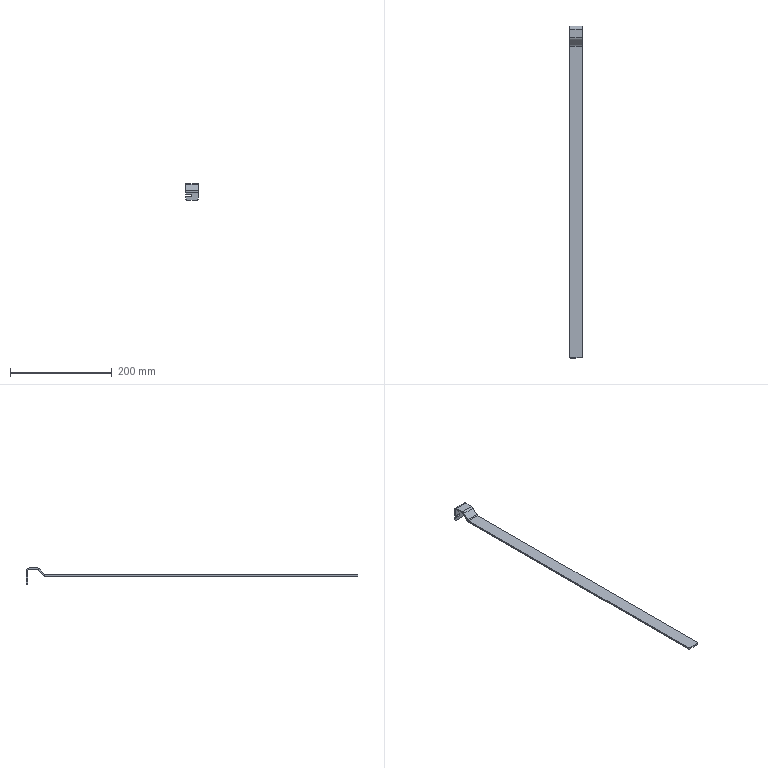Component | SolidWorks | PC-CAJ-P08-1_PM-CAJ-P61-1 | 1 solid | 38 faces | box 25.4 x 651.9 x 31.5 mm | volume 54906 mm3 | plane 28 | cylinder 10 | commonest cylinder face diameters 4 x4 12.7 x3 6.35 x3 | material Plain Carbon Steel
STEP:
#1=COLOUR_RGB('',0.7922,0.8196,0.9333);
#2=FILL_AREA_STYLE_COLOUR('',#1);
#3=FILL_AREA_STYLE('',(#2));
#4=SURFACE_STYLE_FILL_AREA(#3);
#5=SURFACE_SIDE_STYLE('',(#4));
#6=SURFACE_STYLE_USAGE(.BOTH.,#5);
#7=PRESENTATION_STYLE_ASSIGNMENT((#6));
#8=CARTESIAN_POINT('',(0.4213,-26.5,8.548));
#9=VERTEX_POINT('',#8);
#10=CARTESIAN_POINT('',(0.5,-26.421,8.548));
#11=VERTEX_POINT('',#10);
#12=CARTESIAN_POINT('',(0.4213,-26.421,8.548));
#13=DIRECTION('',(0.,0.,1.));
#14=DIRECTION('',(-1.,0.,0.));
#15=AXIS2_PLACEMENT_3D('',#12,#13,#14);
#16=CIRCLE('',#15,0.07874);
#17=EDGE_CURVE('',#9,#11,#16,.T.);
#18=ORIENTED_EDGE('',*,*,#17,.T.);
#19=CARTESIAN_POINT('',(0.5,-26.421,8.673));
#20=VERTEX_POINT('',#19);
#21=CARTESIAN_POINT('',(0.5,-26.421,8.611));
#22=DIRECTION('',(-0.,0.,1.));
#23=VECTOR('',#22,39.37);
#24=LINE('',#21,#23);
#25=EDGE_CURVE('',#11,#20,#24,.T.);
#26=ORIENTED_EDGE('',*,*,#25,.T.);
#27=CARTESIAN_POINT('',(0.4213,-26.5,8.673));
#28=VERTEX_POINT('',#27);
#29=CARTESIAN_POINT('',(0.4213,-26.421,8.673));
#30=DIRECTION('',(-0.,-0.,-1.));
#31=DIRECTION('',(-1.,0.,0.));
#32=AXIS2_PLACEMENT_3D('',#29,#30,#31);
#33=CIRCLE('',#32,0.07874);
#34=EDGE_CURVE('',#20,#28,#33,.T.);
#35=ORIENTED_EDGE('',*,*,#34,.T.);
#36=CARTESIAN_POINT('',(0.4213,-26.5,8.611));
#37=DIRECTION('',(0.,-0.,-1.));
#38=VECTOR('',#37,39.37);
#39=LINE('',#36,#38);
#40=EDGE_CURVE('',#28,#9,#39,.T.);
#41=ORIENTED_EDGE('',*,*,#40,.T.);
#42=EDGE_LOOP('',(#18,#26,#35,#41));
#43=FACE_OUTER_BOUND('',#42,.T.);
#44=CARTESIAN_POINT('',(0.4213,-26.421,8.673));
#45=DIRECTION('',(-0.,-0.,-1.));
#46=DIRECTION('',(-1.,0.,0.));
#47=AXIS2_PLACEMENT_3D('',#44,#45,#46);
#48=CYLINDRICAL_SURFACE('',#47,0.07874);
#49=ADVANCED_FACE('',(#43),#48,.T.);
#50=CARTESIAN_POINT('',(0.5,-2.391,8.548));
#51=VERTEX_POINT('',#50);
#52=CARTESIAN_POINT('',(0.5,-2.391,8.673));
#53=VERTEX_POINT('',#52);
#54=CARTESIAN_POINT('',(0.5,-2.391,8.611));
#55=DIRECTION('',(-0.,0.,1.));
#56=VECTOR('',#55,39.37);
#57=LINE('',#54,#56);
#58=EDGE_CURVE('',#51,#53,#57,.T.);
#59=ORIENTED_EDGE('',*,*,#58,.T.);
#60=CARTESIAN_POINT('',(0.5,-14.406,8.673));
#61=DIRECTION('',(-0.,-1.,0.));
#62=VECTOR('',#61,39.37);
#63=LINE('',#60,#62);
#64=EDGE_CURVE('',#53,#20,#63,.T.);
#65=ORIENTED_EDGE('',*,*,#64,.T.);
#66=ORIENTED_EDGE('',*,*,#25,.F.);
#67=CARTESIAN_POINT('',(0.5,-14.406,8.548));
#68=DIRECTION('',(0.,1.,-0.));
#69=VECTOR('',#68,39.37);
#70=LINE('',#67,#69);
#71=EDGE_CURVE('',#11,#51,#70,.T.);
#72=ORIENTED_EDGE('',*,*,#71,.T.);
#73=EDGE_LOOP('',(#59,#65,#66,#72));
#74=FACE_OUTER_BOUND('',#73,.T.);
#75=CARTESIAN_POINT('',(0.5,-26.421,8.673));
#76=DIRECTION('',(1.,-0.,0.));
#77=DIRECTION('',(0.,-0.,-1.));
#78=AXIS2_PLACEMENT_3D('',#75,#76,#77);
#79=PLANE('',#78);
#80=ADVANCED_FACE('',(#74),#79,.T.);
#81=CARTESIAN_POINT('',(-0.5,-2.391,8.548));
#82=VERTEX_POINT('',#81);
#83=CARTESIAN_POINT('',(0.,-2.391,8.548));
#84=DIRECTION('',(1.,-0.,0.));
#85=VECTOR('',#84,39.37);
#86=LINE('',#83,#85);
#87=EDGE_CURVE('',#82,#51,#86,.T.);
#88=ORIENTED_EDGE('',*,*,#87,.T.);
#89=ORIENTED_EDGE('',*,*,#71,.F.);
#90=ORIENTED_EDGE('',*,*,#17,.F.);
#91=CARTESIAN_POINT('',(-0.4213,-26.5,8.548));
#92=VERTEX_POINT('',#91);
#93=CARTESIAN_POINT('',(-0.,-26.5,8.548));
#94=DIRECTION('',(-1.,0.,-0.));
#95=VECTOR('',#94,39.37);
#96=LINE('',#93,#95);
#97=EDGE_CURVE('',#9,#92,#96,.T.);
#98=ORIENTED_EDGE('',*,*,#97,.T.);
#99=CARTESIAN_POINT('',(-0.5,-26.421,8.548));
#100=VERTEX_POINT('',#99);
#101=CARTESIAN_POINT('',(-0.4213,-26.421,8.548));
#102=DIRECTION('',(0.,-0.,-1.));
#103=DIRECTION('',(-0.,-1.,0.));
#104=AXIS2_PLACEMENT_3D('',#101,#102,#103);
#105=CIRCLE('',#104,0.07874);
#106=EDGE_CURVE('',#92,#100,#105,.T.);
#107=ORIENTED_EDGE('',*,*,#106,.T.);
#108=CARTESIAN_POINT('',(-0.5,-14.445,8.548));
#109=DIRECTION('',(0.,1.,-0.));
#110=VECTOR('',#109,39.37);
#111=LINE('',#108,#110);
#112=EDGE_CURVE('',#100,#82,#111,.T.);
#113=ORIENTED_EDGE('',*,*,#112,.T.);
#114=EDGE_LOOP('',(#88,#89,#90,#98,#107,#113));
#115=FACE_OUTER_BOUND('',#114,.T.);
#116=CARTESIAN_POINT('',(0.5,-2.391,8.548));
#117=DIRECTION('',(0.,-0.,-1.));
#118=DIRECTION('',(-0.,-1.,0.));
#119=AXIS2_PLACEMENT_3D('',#116,#117,#118);
#120=PLANE('',#119);
#121=ADVANCED_FACE('',(#115),#120,.T.);
#122=CARTESIAN_POINT('',(-0.4213,-26.5,8.673));
#123=VERTEX_POINT('',#122);
#124=CARTESIAN_POINT('',(-0.4213,-26.5,8.611));
#125=DIRECTION('',(0.,-0.,-1.));
#126=VECTOR('',#125,39.37);
#127=LINE('',#124,#126);
#128=EDGE_CURVE('',#123,#92,#127,.T.);
#129=ORIENTED_EDGE('',*,*,#128,.T.);
#130=ORIENTED_EDGE('',*,*,#97,.F.);
#131=ORIENTED_EDGE('',*,*,#40,.F.);
#132=CARTESIAN_POINT('',(-0.,-26.5,8.673));
#133=DIRECTION('',(-1.,0.,-0.));
#134=VECTOR('',#133,39.37);
#135=LINE('',#132,#134);
#136=EDGE_CURVE('',#28,#123,#135,.T.);
#137=ORIENTED_EDGE('',*,*,#136,.T.);
#138=EDGE_LOOP('',(#129,#130,#131,#137));
#139=FACE_OUTER_BOUND('',#138,.T.);
#140=CARTESIAN_POINT('',(0.4213,-26.5,8.548));
#141=DIRECTION('',(-0.,-1.,0.));
#142=DIRECTION('',(-0.,0.,1.));
#143=AXIS2_PLACEMENT_3D('',#140,#141,#142);
#144=PLANE('',#143);
#145=ADVANCED_FACE('',(#139),#144,.T.);
#146=CARTESIAN_POINT('',(-0.5,-26.421,8.673));
#147=VERTEX_POINT('',#146);
#148=CARTESIAN_POINT('',(-0.4213,-26.421,8.673));
#149=DIRECTION('',(-0.,0.,1.));
#150=DIRECTION('',(-0.,-1.,0.));
#151=AXIS2_PLACEMENT_3D('',#148,#149,#150);
#152=CIRCLE('',#151,0.07874);
#153=EDGE_CURVE('',#147,#123,#152,.T.);
#154=ORIENTED_EDGE('',*,*,#153,.T.);
#155=ORIENTED_EDGE('',*,*,#136,.F.);
#156=ORIENTED_EDGE('',*,*,#34,.F.);
#157=ORIENTED_EDGE('',*,*,#64,.F.);
#158=CARTESIAN_POINT('',(-0.5,-2.391,8.673));
#159=VERTEX_POINT('',#158);
#160=CARTESIAN_POINT('',(0.,-2.391,8.673));
#161=DIRECTION('',(-1.,0.,-0.));
#162=VECTOR('',#161,39.37);
#163=LINE('',#160,#162);
#164=EDGE_CURVE('',#53,#159,#163,.T.);
#165=ORIENTED_EDGE('',*,*,#164,.T.);
#166=CARTESIAN_POINT('',(-0.5,-14.445,8.673));
#167=DIRECTION('',(-0.,-1.,0.));
#168=VECTOR('',#167,39.37);
#169=LINE('',#166,#168);
#170=EDGE_CURVE('',#159,#147,#169,.T.);
#171=ORIENTED_EDGE('',*,*,#170,.T.);
#172=EDGE_LOOP('',(#154,#155,#156,#157,#165,#171));
#173=FACE_OUTER_BOUND('',#172,.T.);
#174=CARTESIAN_POINT('',(0.5,-26.5,8.673));
#175=DIRECTION('',(-0.,0.,1.));
#176=DIRECTION('',(0.,1.,-0.));
#177=AXIS2_PLACEMENT_3D('',#174,#175,#176);
#178=PLANE('',#177);
#179=ADVANCED_FACE('',(#173),#178,.T.);
#180=ORIENTED_EDGE('',*,*,#58,.F.);
#181=CARTESIAN_POINT('',(0.5,-2.214,8.621));
#182=VERTEX_POINT('',#181);
#183=CARTESIAN_POINT('',(0.5,-2.391,8.798));
#184=DIRECTION('',(1.,-0.,-0.));
#185=DIRECTION('',(0.,0.,1.));
#186=AXIS2_PLACEMENT_3D('',#183,#184,#185);
#187=CIRCLE('',#186,0.25);
#188=EDGE_CURVE('',#51,#182,#187,.T.);
#189=ORIENTED_EDGE('',*,*,#188,.T.);
#190=CARTESIAN_POINT('',(0.5,-2.303,8.71));
#191=VERTEX_POINT('',#190);
#192=CARTESIAN_POINT('',(0.5,-2.214,8.621));
#193=DIRECTION('',(-0.,-0.7071,0.7071));
#194=VECTOR('',#193,39.37);
#195=LINE('',#192,#194);
#196=EDGE_CURVE('',#182,#191,#195,.T.);
#197=ORIENTED_EDGE('',*,*,#196,.T.);
#198=CARTESIAN_POINT('',(0.5,-2.391,8.798));
#199=DIRECTION('',(-1.,0.,-0.));
#200=DIRECTION('',(0.,-0.,-1.));
#201=AXIS2_PLACEMENT_3D('',#198,#199,#200);
#202=CIRCLE('',#201,0.125);
#203=EDGE_CURVE('',#191,#53,#202,.T.);
#204=ORIENTED_EDGE('',*,*,#203,.T.);
#205=EDGE_LOOP('',(#180,#189,#197,#204));
#206=FACE_OUTER_BOUND('',#205,.T.);
#207=CARTESIAN_POINT('',(0.5,-2.391,8.71));
#208=DIRECTION('',(1.,-0.,0.));
#209=DIRECTION('',(0.,-0.,-1.));
#210=AXIS2_PLACEMENT_3D('',#207,#208,#209);
#211=PLANE('',#210);
#212=ADVANCED_FACE('',(#206),#211,.T.);
#213=ORIENTED_EDGE('',*,*,#87,.F.);
#214=CARTESIAN_POINT('',(-0.5,-2.214,8.621));
#215=VERTEX_POINT('',#214);
#216=CARTESIAN_POINT('',(-0.5,-2.391,8.798));
#217=DIRECTION('',(1.,-0.,-0.));
#218=DIRECTION('',(0.,0.,1.));
#219=AXIS2_PLACEMENT_3D('',#216,#217,#218);
#220=CIRCLE('',#219,0.25);
#221=EDGE_CURVE('',#82,#215,#220,.T.);
#222=ORIENTED_EDGE('',*,*,#221,.T.);
#223=CARTESIAN_POINT('',(0.,-2.214,8.621));
#224=DIRECTION('',(1.,-0.,0.));
#225=VECTOR('',#224,39.37);
#226=LINE('',#223,#225);
#227=EDGE_CURVE('',#215,#182,#226,.T.);
#228=ORIENTED_EDGE('',*,*,#227,.T.);
#229=ORIENTED_EDGE('',*,*,#188,.F.);
#230=EDGE_LOOP('',(#213,#222,#228,#229));
#231=FACE_OUTER_BOUND('',#230,.T.);
#232=CARTESIAN_POINT('',(0.5,-2.391,8.798));
#233=DIRECTION('',(-1.,0.,0.));
#234=DIRECTION('',(0.,0.,1.));
#235=AXIS2_PLACEMENT_3D('',#232,#233,#234);
#236=CYLINDRICAL_SURFACE('',#235,0.25);
#237=ADVANCED_FACE('',(#231),#236,.T.);
#238=CARTESIAN_POINT('',(-0.5,-2.391,8.611));
#239=DIRECTION('',(0.,-0.,-1.));
#240=VECTOR('',#239,39.37);
#241=LINE('',#238,#240);
#242=EDGE_CURVE('',#159,#82,#241,.T.);
#243=ORIENTED_EDGE('',*,*,#242,.T.);
#244=ORIENTED_EDGE('',*,*,#112,.F.);
#245=CARTESIAN_POINT('',(-0.5,-26.421,8.611));
#246=DIRECTION('',(-0.,0.,1.));
#247=VECTOR('',#246,39.37);
#248=LINE('',#245,#247);
#249=EDGE_CURVE('',#100,#147,#248,.T.);
#250=ORIENTED_EDGE('',*,*,#249,.T.);
#251=ORIENTED_EDGE('',*,*,#170,.F.);
#252=EDGE_LOOP('',(#243,#244,#250,#251));
#253=FACE_OUTER_BOUND('',#252,.T.);
#254=CARTESIAN_POINT('',(-0.5,-26.421,8.548));
#255=DIRECTION('',(-1.,0.,-0.));
#256=DIRECTION('',(-0.,0.,1.));
#257=AXIS2_PLACEMENT_3D('',#254,#255,#256);
#258=PLANE('',#257);
#259=ADVANCED_FACE('',(#253),#258,.T.);
#260=ORIENTED_EDGE('',*,*,#106,.F.);
#261=ORIENTED_EDGE('',*,*,#128,.F.);
#262=ORIENTED_EDGE('',*,*,#153,.F.);
#263=ORIENTED_EDGE('',*,*,#249,.F.);
#264=EDGE_LOOP('',(#260,#261,#262,#263));
#265=FACE_OUTER_BOUND('',#264,.T.);
#266=CARTESIAN_POINT('',(-0.4213,-26.421,8.673));
#267=DIRECTION('',(0.,-0.,-1.));
#268=DIRECTION('',(-0.,-1.,0.));
#269=AXIS2_PLACEMENT_3D('',#266,#267,#268);
#270=CYLINDRICAL_SURFACE('',#269,0.07874);
#271=ADVANCED_FACE('',(#265),#270,.T.);
#272=ORIENTED_EDGE('',*,*,#164,.F.);
#273=ORIENTED_EDGE('',*,*,#203,.F.);
#274=CARTESIAN_POINT('',(-0.5,-2.303,8.71));
#275=VERTEX_POINT('',#274);
#276=CARTESIAN_POINT('',(0.,-2.303,8.71));
#277=DIRECTION('',(-1.,0.,-0.));
#278=VECTOR('',#277,39.37);
#279=LINE('',#276,#278);
#280=EDGE_CURVE('',#191,#275,#279,.T.);
#281=ORIENTED_EDGE('',*,*,#280,.T.);
#282=CARTESIAN_POINT('',(-0.5,-2.391,8.798));
#283=DIRECTION('',(-1.,0.,-0.));
#284=DIRECTION('',(0.,-0.,-1.));
#285=AXIS2_PLACEMENT_3D('',#282,#283,#284);
#286=CIRCLE('',#285,0.125);
#287=EDGE_CURVE('',#275,#159,#286,.T.);
#288=ORIENTED_EDGE('',*,*,#287,.T.);
#289=EDGE_LOOP('',(#272,#273,#281,#288));
#290=FACE_OUTER_BOUND('',#289,.T.);
#291=CARTESIAN_POINT('',(-0.5,-2.391,8.798));
#292=DIRECTION('',(1.,-0.,0.));
#293=DIRECTION('',(0.,-0.,-1.));
#294=AXIS2_PLACEMENT_3D('',#291,#292,#293);
#295=CYLINDRICAL_SURFACE('',#294,0.125);
#296=ADVANCED_FACE('',(#290),#295,.F.);
#297=ORIENTED_EDGE('',*,*,#196,.F.);
#298=CARTESIAN_POINT('',(0.5,-1.804,9.032));
#299=VERTEX_POINT('',#298);
#300=CARTESIAN_POINT('',(0.5,-2.009,8.827));
#301=DIRECTION('',(0.,0.7071,0.7071));
#302=VECTOR('',#301,39.37);
#303=LINE('',#300,#302);
#304=EDGE_CURVE('',#182,#299,#303,.T.);
#305=ORIENTED_EDGE('',*,*,#304,.T.);
#306=CARTESIAN_POINT('',(0.5,-1.892,9.12));
#307=VERTEX_POINT('',#306);
#308=CARTESIAN_POINT('',(0.5,-1.848,9.076));
#309=DIRECTION('',(-0.,-0.7071,0.7071));
#310=VECTOR('',#309,39.37);
#311=LINE('',#308,#310);
#312=EDGE_CURVE('',#299,#307,#311,.T.);
#313=ORIENTED_EDGE('',*,*,#312,.T.);
#314=CARTESIAN_POINT('',(0.5,-2.097,8.915));
#315=DIRECTION('',(-0.,-0.7071,-0.7071));
#316=VECTOR('',#315,39.37);
#317=LINE('',#314,#316);
#318=EDGE_CURVE('',#307,#191,#317,.T.);
#319=ORIENTED_EDGE('',*,*,#318,.T.);
#320=EDGE_LOOP('',(#297,#305,#313,#319));
#321=FACE_OUTER_BOUND('',#320,.T.);
#322=CARTESIAN_POINT('',(0.5,-2.552,8.871));
#323=DIRECTION('',(1.,-0.,0.));
#324=DIRECTION('',(0.,0.7071,-0.7071));
#325=AXIS2_PLACEMENT_3D('',#322,#323,#324);
#326=PLANE('',#325);
#327=ADVANCED_FACE('',(#321),#326,.T.);
#328=ORIENTED_EDGE('',*,*,#242,.F.);
#329=ORIENTED_EDGE('',*,*,#287,.F.);
#330=CARTESIAN_POINT('',(-0.5,-2.303,8.71));
#331=DIRECTION('',(0.,0.7071,-0.7071));
#332=VECTOR('',#331,39.37);
#333=LINE('',#330,#332);
#334=EDGE_CURVE('',#275,#215,#333,.T.);
#335=ORIENTED_EDGE('',*,*,#334,.T.);
#336=ORIENTED_EDGE('',*,*,#221,.F.);
#337=EDGE_LOOP('',(#328,#329,#335,#336));
#338=FACE_OUTER_BOUND('',#337,.T.);
#339=CARTESIAN_POINT('',(-0.5,-2.391,8.548));
#340=DIRECTION('',(-1.,0.,-0.));
#341=DIRECTION('',(-0.,0.,1.));
#342=AXIS2_PLACEMENT_3D('',#339,#340,#341);
#343=PLANE('',#342);
#344=ADVANCED_FACE('',(#338),#343,.T.);
#345=ORIENTED_EDGE('',*,*,#227,.F.);
#346=CARTESIAN_POINT('',(-0.5,-1.804,9.032));
#347=VERTEX_POINT('',#346);
#348=CARTESIAN_POINT('',(-0.5,-2.009,8.827));
#349=DIRECTION('',(0.,0.7071,0.7071));
#350=VECTOR('',#349,39.37);
#351=LINE('',#348,#350);
#352=EDGE_CURVE('',#215,#347,#351,.T.);
#353=ORIENTED_EDGE('',*,*,#352,.T.);
#354=CARTESIAN_POINT('',(0.,-1.804,9.032));
#355=DIRECTION('',(1.,-0.,0.));
#356=VECTOR('',#355,39.37);
#357=LINE('',#354,#356);
#358=EDGE_CURVE('',#347,#299,#357,.T.);
#359=ORIENTED_EDGE('',*,*,#358,.T.);
#360=ORIENTED_EDGE('',*,*,#304,.F.);
#361=EDGE_LOOP('',(#345,#353,#359,#360));
#362=FACE_OUTER_BOUND('',#361,.T.);
#363=CARTESIAN_POINT('',(0.5,-1.804,9.032));
#364=DIRECTION('',(0.,0.7071,-0.7071));
#365=DIRECTION('',(-0.,-0.7071,-0.7071));
#366=AXIS2_PLACEMENT_3D('',#363,#364,#365);
#367=PLANE('',#366);
#368=ADVANCED_FACE('',(#362),#367,.T.);
#369=ORIENTED_EDGE('',*,*,#280,.F.);
#370=ORIENTED_EDGE('',*,*,#318,.F.);
#371=CARTESIAN_POINT('',(-0.5,-1.892,9.12));
#372=VERTEX_POINT('',#371);
#373=CARTESIAN_POINT('',(0.,-1.892,9.12));
#374=DIRECTION('',(-1.,0.,-0.));
#375=VECTOR('',#374,39.37);
#376=LINE('',#373,#375);
#377=EDGE_CURVE('',#307,#372,#376,.T.);
#378=ORIENTED_EDGE('',*,*,#377,.T.);
#379=CARTESIAN_POINT('',(-0.5,-2.097,8.915));
#380=DIRECTION('',(-0.,-0.7071,-0.7071));
#381=VECTOR('',#380,39.37);
#382=LINE('',#379,#381);
#383=EDGE_CURVE('',#372,#275,#382,.T.);
#384=ORIENTED_EDGE('',*,*,#383,.T.);
#385=EDGE_LOOP('',(#369,#370,#378,#384));
#386=FACE_OUTER_BOUND('',#385,.T.);
#387=CARTESIAN_POINT('',(0.5,-2.303,8.71));
#388=DIRECTION('',(-0.,-0.7071,0.7071));
#389=DIRECTION('',(0.,0.7071,0.7071));
#390=AXIS2_PLACEMENT_3D('',#387,#388,#389);
#391=PLANE('',#390);
#392=ADVANCED_FACE('',(#386),#391,.T.);
#393=ORIENTED_EDGE('',*,*,#312,.F.);
#394=CARTESIAN_POINT('',(0.5,-1.715,9.068));
#395=VERTEX_POINT('',#394);
#396=CARTESIAN_POINT('',(0.5,-1.715,8.943));
#397=DIRECTION('',(-1.,0.,-0.));
#398=DIRECTION('',(-0.,0.,1.));
#399=AXIS2_PLACEMENT_3D('',#396,#397,#398);
#400=CIRCLE('',#399,0.125);
#401=EDGE_CURVE('',#299,#395,#400,.T.);
#402=ORIENTED_EDGE('',*,*,#401,.T.);
#403=CARTESIAN_POINT('',(0.5,-1.715,9.193));
#404=VERTEX_POINT('',#403);
#405=CARTESIAN_POINT('',(0.5,-1.715,9.113));
#406=DIRECTION('',(-0.,0.,1.));
#407=VECTOR('',#406,39.37);
#408=LINE('',#405,#407);
#409=EDGE_CURVE('',#395,#404,#408,.T.);
#410=ORIENTED_EDGE('',*,*,#409,.T.);
#411=CARTESIAN_POINT('',(0.5,-1.715,8.943));
#412=DIRECTION('',(1.,-0.,-0.));
#413=DIRECTION('',(-0.,-0.,-1.));
#414=AXIS2_PLACEMENT_3D('',#411,#412,#413);
#415=CIRCLE('',#414,0.25);
#416=EDGE_CURVE('',#404,#307,#415,.T.);
#417=ORIENTED_EDGE('',*,*,#416,.T.);
#418=EDGE_LOOP('',(#393,#402,#410,#417));
#419=FACE_OUTER_BOUND('',#418,.T.);
#420=CARTESIAN_POINT('',(0.5,-1.892,9.193));
#421=DIRECTION('',(1.,-0.,0.));
#422=DIRECTION('',(0.,-0.,-1.));
#423=AXIS2_PLACEMENT_3D('',#420,#421,#422);
#424=PLANE('',#423);
#425=ADVANCED_FACE('',(#419),#424,.T.);
#426=ORIENTED_EDGE('',*,*,#334,.F.);
#427=ORIENTED_EDGE('',*,*,#383,.F.);
#428=CARTESIAN_POINT('',(-0.5,-1.848,9.076));
#429=DIRECTION('',(0.,0.7071,-0.7071));
#430=VECTOR('',#429,39.37);
#431=LINE('',#428,#430);
#432=EDGE_CURVE('',#372,#347,#431,.T.);
#433=ORIENTED_EDGE('',*,*,#432,.T.);
#434=ORIENTED_EDGE('',*,*,#352,.F.);
#435=EDGE_LOOP('',(#426,#427,#433,#434));
#436=FACE_OUTER_BOUND('',#435,.T.);
#437=CARTESIAN_POINT('',(-0.5,-2.053,8.372));
#438=DIRECTION('',(-1.,0.,-0.));
#439=DIRECTION('',(-0.,-0.7071,0.7071));
#440=AXIS2_PLACEMENT_3D('',#437,#438,#439);
#441=PLANE('',#440);
#442=ADVANCED_FACE('',(#436),#441,.T.);
#443=ORIENTED_EDGE('',*,*,#358,.F.);
#444=CARTESIAN_POINT('',(-0.5,-1.715,9.068));
#445=VERTEX_POINT('',#444);
#446=CARTESIAN_POINT('',(-0.5,-1.715,8.943));
#447=DIRECTION('',(-1.,0.,-0.));
#448=DIRECTION('',(-0.,0.,1.));
#449=AXIS2_PLACEMENT_3D('',#446,#447,#448);
#450=CIRCLE('',#449,0.125);
#451=EDGE_CURVE('',#347,#445,#450,.T.);
#452=ORIENTED_EDGE('',*,*,#451,.T.);
#453=CARTESIAN_POINT('',(0.,-1.715,9.068));
#454=DIRECTION('',(1.,-0.,0.));
#455=VECTOR('',#454,39.37);
#456=LINE('',#453,#455);
#457=EDGE_CURVE('',#445,#395,#456,.T.);
#458=ORIENTED_EDGE('',*,*,#457,.T.);
#459=ORIENTED_EDGE('',*,*,#401,.F.);
#460=EDGE_LOOP('',(#443,#452,#458,#459));
#461=FACE_OUTER_BOUND('',#460,.T.);
#462=CARTESIAN_POINT('',(0.5,-1.715,8.943));
#463=DIRECTION('',(-1.,0.,-0.));
#464=DIRECTION('',(-0.,0.,1.));
#465=AXIS2_PLACEMENT_3D('',#462,#463,#464);
#466=CYLINDRICAL_SURFACE('',#465,0.125);
#467=ADVANCED_FACE('',(#461),#466,.F.);
#468=ORIENTED_EDGE('',*,*,#377,.F.);
#469=ORIENTED_EDGE('',*,*,#416,.F.);
#470=CARTESIAN_POINT('',(-0.5,-1.715,9.193));
#471=VERTEX_POINT('',#470);
#472=CARTESIAN_POINT('',(0.,-1.715,9.193));
#473=DIRECTION('',(-1.,0.,-0.));
#474=VECTOR('',#473,39.37);
#475=LINE('',#472,#474);
#476=EDGE_CURVE('',#404,#471,#475,.T.);
#477=ORIENTED_EDGE('',*,*,#476,.T.);
#478=CARTESIAN_POINT('',(-0.5,-1.715,8.943));
#479=DIRECTION('',(1.,-0.,-0.));
#480=DIRECTION('',(-0.,-0.,-1.));
#481=AXIS2_PLACEMENT_3D('',#478,#479,#480);
#482=CIRCLE('',#481,0.25);
#483=EDGE_CURVE('',#471,#372,#482,.T.);
#484=ORIENTED_EDGE('',*,*,#483,.T.);
#485=EDGE_LOOP('',(#468,#469,#477,#484));
#486=FACE_OUTER_BOUND('',#485,.T.);
#487=CARTESIAN_POINT('',(-0.5,-1.715,8.943));
#488=DIRECTION('',(1.,-0.,-0.));
#489=DIRECTION('',(-0.,-0.,-1.));
#490=AXIS2_PLACEMENT_3D('',#487,#488,#489);
#491=CYLINDRICAL_SURFACE('',#490,0.25);
#492=ADVANCED_FACE('',(#486),#491,.T.);
#493=ORIENTED_EDGE('',*,*,#409,.F.);
#494=CARTESIAN_POINT('',(0.5,-1.085,9.068));
#495=VERTEX_POINT('',#494);
#496=CARTESIAN_POINT('',(0.5,-1.715,9.068));
#497=DIRECTION('',(0.,1.,-0.));
#498=VECTOR('',#497,39.37);
#499=LINE('',#496,#498);
#500=EDGE_CURVE('',#395,#495,#499,.T.);
#501=ORIENTED_EDGE('',*,*,#500,.T.);
#502=CARTESIAN_POINT('',(0.5,-1.085,9.193));
#503=VERTEX_POINT('',#502);
#504=CARTESIAN_POINT('',(0.5,-1.085,9.068));
#505=DIRECTION('',(-0.,-0.,1.));
#506=VECTOR('',#505,39.37);
#507=LINE('',#504,#506);
#508=EDGE_CURVE('',#495,#503,#507,.T.);
#509=ORIENTED_EDGE('',*,*,#508,.T.);
#510=CARTESIAN_POINT('',(0.5,-1.085,9.193));
#511=DIRECTION('',(-0.,-1.,0.));
#512=VECTOR('',#511,39.37);
#513=LINE('',#510,#512);
#514=EDGE_CURVE('',#503,#404,#513,.T.);
#515=ORIENTED_EDGE('',*,*,#514,.T.);
#516=EDGE_LOOP('',(#493,#501,#509,#515));
#517=FACE_OUTER_BOUND('',#516,.T.);
#518=CARTESIAN_POINT('',(0.5,-1.4,9.509));
#519=DIRECTION('',(1.,-0.,0.));
#520=DIRECTION('',(-0.,-0.7071,-0.7071));
#521=AXIS2_PLACEMENT_3D('',#518,#519,#520);
#522=PLANE('',#521);
#523=ADVANCED_FACE('',(#517),#522,.T.);
#524=ORIENTED_EDGE('',*,*,#432,.F.);
#525=ORIENTED_EDGE('',*,*,#483,.F.);
#526=CARTESIAN_POINT('',(-0.5,-1.715,9.113));
#527=DIRECTION('',(0.,-0.,-1.));
#528=VECTOR('',#527,39.37);
#529=LINE('',#526,#528);
#530=EDGE_CURVE('',#471,#445,#529,.T.);
#531=ORIENTED_EDGE('',*,*,#530,.T.);
#532=ORIENTED_EDGE('',*,*,#451,.F.);
#533=EDGE_LOOP('',(#524,#525,#531,#532));
#534=FACE_OUTER_BOUND('',#533,.T.);
#535=CARTESIAN_POINT('',(-0.5,-1.892,9.032));
#536=DIRECTION('',(-1.,0.,-0.));
#537=DIRECTION('',(-0.,0.,1.));
#538=AXIS2_PLACEMENT_3D('',#535,#536,#537);
#539=PLANE('',#538);
#540=ADVANCED_FACE('',(#534),#539,.T.);
#541=ORIENTED_EDGE('',*,*,#457,.F.);
#542=CARTESIAN_POINT('',(-0.5,-1.085,9.068));
#543=VERTEX_POINT('',#542);
#544=CARTESIAN_POINT('',(-0.5,-1.4,9.068));
#545=DIRECTION('',(0.,1.,0.));
#546=VECTOR('',#545,39.37);
#547=LINE('',#544,#546);
#548=EDGE_CURVE('',#445,#543,#547,.T.);
#549=ORIENTED_EDGE('',*,*,#548,.T.);
#550=CARTESIAN_POINT('',(0.,-1.085,9.068));
#551=DIRECTION('',(1.,-0.,0.));
#552=VECTOR('',#551,39.37);
#553=LINE('',#550,#552);
#554=EDGE_CURVE('',#543,#495,#553,.T.);
#555=ORIENTED_EDGE('',*,*,#554,.T.);
#556=ORIENTED_EDGE('',*,*,#500,.F.);
#557=EDGE_LOOP('',(#541,#549,#555,#556));
#558=FACE_OUTER_BOUND('',#557,.T.);
#559=CARTESIAN_POINT('',(0.5,-1.085,9.068));
#560=DIRECTION('',(0.,0.,-1.));
#561=DIRECTION('',(-0.,-1.,-0.));
#562=AXIS2_PLACEMENT_3D('',#559,#560,#561);
#563=PLANE('',#562);
#564=ADVANCED_FACE('',(#558),#563,.T.);
#565=ORIENTED_EDGE('',*,*,#476,.F.);
#566=ORIENTED_EDGE('',*,*,#514,.F.);
#567=CARTESIAN_POINT('',(-0.5,-1.085,9.193));
#568=VERTEX_POINT('',#567);
#569=CARTESIAN_POINT('',(0.,-1.085,9.193));
#570=DIRECTION('',(-1.,0.,-0.));
#571=VECTOR('',#570,39.37);
#572=LINE('',#569,#571);
#573=EDGE_CURVE('',#503,#568,#572,.T.);
#574=ORIENTED_EDGE('',*,*,#573,.T.);
#575=CARTESIAN_POINT('',(-0.5,-1.4,9.193));
#576=DIRECTION('',(-0.,-1.,-0.));
#577=VECTOR('',#576,39.37);
#578=LINE('',#575,#577);
#579=EDGE_CURVE('',#568,#471,#578,.T.);
#580=ORIENTED_EDGE('',*,*,#579,.T.);
#581=EDGE_LOOP('',(#565,#566,#574,#580));
#582=FACE_OUTER_BOUND('',#581,.T.);
#583=CARTESIAN_POINT('',(0.5,-1.715,9.193));
#584=DIRECTION('',(-0.,-0.,1.));
#585=DIRECTION('',(0.,1.,0.));
#586=AXIS2_PLACEMENT_3D('',#583,#584,#585);
#587=PLANE('',#586);
#588=ADVANCED_FACE('',(#582),#587,.T.);
#589=ORIENTED_EDGE('',*,*,#508,.F.);
#590=CARTESIAN_POINT('',(0.5,-0.9598,8.943));
#591=VERTEX_POINT('',#590);
#592=CARTESIAN_POINT('',(0.5,-1.085,8.943));
#593=DIRECTION('',(-1.,0.,-0.));
#594=DIRECTION('',(-0.,0.,1.));
#595=AXIS2_PLACEMENT_3D('',#592,#593,#594);
#596=CIRCLE('',#595,0.125);
#597=EDGE_CURVE('',#495,#591,#596,.T.);
#598=ORIENTED_EDGE('',*,*,#597,.T.);
#599=CARTESIAN_POINT('',(0.5,-0.8348,8.943));
#600=VERTEX_POINT('',#599);
#601=CARTESIAN_POINT('',(0.5,-0.9598,8.943));
#602=DIRECTION('',(0.,1.,-0.));
#603=VECTOR('',#602,39.37);
#604=LINE('',#601,#603);
#605=EDGE_CURVE('',#591,#600,#604,.T.);
#606=ORIENTED_EDGE('',*,*,#605,.T.);
#607=CARTESIAN_POINT('',(0.5,-1.085,8.943));
#608=DIRECTION('',(1.,-0.,-0.));
#609=DIRECTION('',(0.,-0.,-1.));
#610=AXIS2_PLACEMENT_3D('',#607,#608,#609);
#611=CIRCLE('',#610,0.25);
#612=EDGE_CURVE('',#600,#503,#611,.T.);
#613=ORIENTED_EDGE('',*,*,#612,.T.);
#614=EDGE_LOOP('',(#589,#598,#606,#613));
#615=FACE_OUTER_BOUND('',#614,.T.);
#616=CARTESIAN_POINT('',(0.5,-1.085,9.193));
#617=DIRECTION('',(1.,-0.,0.));
#618=DIRECTION('',(0.,-0.,-1.));
#619=AXIS2_PLACEMENT_3D('',#616,#617,#618);
#620=PLANE('',#619);
#621=ADVANCED_FACE('',(#615),#620,.T.);
#622=ORIENTED_EDGE('',*,*,#530,.F.);
#623=ORIENTED_EDGE('',*,*,#579,.F.);
#624=CARTESIAN_POINT('',(-0.5,-1.085,9.193));
#625=DIRECTION('',(0.,0.,-1.));
#626=VECTOR('',#625,39.37);
#627=LINE('',#624,#626);
#628=EDGE_CURVE('',#568,#543,#627,.T.);
#629=ORIENTED_EDGE('',*,*,#628,.T.);
#630=ORIENTED_EDGE('',*,*,#548,.F.);
#631=EDGE_LOOP('',(#622,#623,#629,#630));
#632=FACE_OUTER_BOUND('',#631,.T.);
#633=CARTESIAN_POINT('',(-0.5,-1.778,9.131));
#634=DIRECTION('',(-1.,0.,-0.));
#635=DIRECTION('',(0.,0.7071,0.7071));
#636=AXIS2_PLACEMENT_3D('',#633,#634,#635);
#637=PLANE('',#636);
#638=ADVANCED_FACE('',(#632),#637,.T.);
#639=ORIENTED_EDGE('',*,*,#554,.F.);
#640=CARTESIAN_POINT('',(-0.5,-0.9598,8.943));
#641=VERTEX_POINT('',#640);
#642=CARTESIAN_POINT('',(-0.5,-1.085,8.943));
#643=DIRECTION('',(-1.,0.,-0.));
#644=DIRECTION('',(-0.,0.,1.));
#645=AXIS2_PLACEMENT_3D('',#642,#643,#644);
#646=CIRCLE('',#645,0.125);
#647=EDGE_CURVE('',#543,#641,#646,.T.);
#648=ORIENTED_EDGE('',*,*,#647,.T.);
#649=CARTESIAN_POINT('',(0.,-0.9598,8.943));
#650=DIRECTION('',(1.,-0.,0.));
#651=VECTOR('',#650,39.37);
#652=LINE('',#649,#651);
#653=EDGE_CURVE('',#641,#591,#652,.T.);
#654=ORIENTED_EDGE('',*,*,#653,.T.);
#655=ORIENTED_EDGE('',*,*,#597,.F.);
#656=EDGE_LOOP('',(#639,#648,#654,#655));
#657=FACE_OUTER_BOUND('',#656,.T.);
#658=CARTESIAN_POINT('',(0.5,-1.085,8.943));
#659=DIRECTION('',(-1.,0.,-0.));
#660=DIRECTION('',(-0.,0.,1.));
#661=AXIS2_PLACEMENT_3D('',#658,#659,#660);
#662=CYLINDRICAL_SURFACE('',#661,0.125);
#663=ADVANCED_FACE('',(#657),#662,.F.);
#664=ORIENTED_EDGE('',*,*,#573,.F.);
#665=ORIENTED_EDGE('',*,*,#612,.F.);
#666=CARTESIAN_POINT('',(-0.5,-0.8348,8.943));
#667=VERTEX_POINT('',#666);
#668=CARTESIAN_POINT('',(0.,-0.8348,8.943));
#669=DIRECTION('',(-1.,0.,-0.));
#670=VECTOR('',#669,39.37);
#671=LINE('',#668,#670);
#672=EDGE_CURVE('',#600,#667,#671,.T.);
#673=ORIENTED_EDGE('',*,*,#672,.T.);
#674=CARTESIAN_POINT('',(-0.5,-1.085,8.943));
#675=DIRECTION('',(1.,-0.,-0.));
#676=DIRECTION('',(0.,-0.,-1.));
#677=AXIS2_PLACEMENT_3D('',#674,#675,#676);
#678=CIRCLE('',#677,0.25);
#679=EDGE_CURVE('',#667,#568,#678,.T.);
#680=ORIENTED_EDGE('',*,*,#679,.T.);
#681=EDGE_LOOP('',(#664,#665,#673,#680));
#682=FACE_OUTER_BOUND('',#681,.T.);
#683=CARTESIAN_POINT('',(-0.5,-1.085,8.943));
#684=DIRECTION('',(1.,-0.,-0.));
#685=DIRECTION('',(0.,-0.,-1.));
#686=AXIS2_PLACEMENT_3D('',#683,#684,#685);
#687=CYLINDRICAL_SURFACE('',#686,0.25);
#688=ADVANCED_FACE('',(#682),#687,.T.);
#689=ORIENTED_EDGE('',*,*,#605,.F.);
#690=CARTESIAN_POINT('',(0.5,-0.9598,8.032));
#691=VERTEX_POINT('',#690);
#692=CARTESIAN_POINT('',(0.5,-0.9598,8.488));
#693=DIRECTION('',(0.,-0.,-1.));
#694=VECTOR('',#693,39.37);
#695=LINE('',#692,#694);
#696=EDGE_CURVE('',#591,#691,#695,.T.);
#697=ORIENTED_EDGE('',*,*,#696,.T.);
#698=CARTESIAN_POINT('',(0.5,-0.8348,8.032));
#699=VERTEX_POINT('',#698);
#700=CARTESIAN_POINT('',(0.5,-0.8973,8.032));
#701=DIRECTION('',(0.,1.,-0.));
#702=VECTOR('',#701,39.37);
#703=LINE('',#700,#702);
#704=EDGE_CURVE('',#691,#699,#703,.T.);
#705=ORIENTED_EDGE('',*,*,#704,.T.);
#706=CARTESIAN_POINT('',(0.5,-0.8348,8.488));
#707=DIRECTION('',(-0.,0.,1.));
#708=VECTOR('',#707,39.37);
#709=LINE('',#706,#708);
#710=EDGE_CURVE('',#699,#600,#709,.T.);
#711=ORIENTED_EDGE('',*,*,#710,.T.);
#712=EDGE_LOOP('',(#689,#697,#705,#711));
#713=FACE_OUTER_BOUND('',#712,.T.);
#714=CARTESIAN_POINT('',(0.5,-0.8348,8.943));
#715=DIRECTION('',(1.,-0.,0.));
#716=DIRECTION('',(-0.,-1.,-0.));
#717=AXIS2_PLACEMENT_3D('',#714,#715,#716);
#718=PLANE('',#717);
#719=ADVANCED_FACE('',(#713),#718,.T.);
#720=ORIENTED_EDGE('',*,*,#628,.F.);
#721=ORIENTED_EDGE('',*,*,#679,.F.);
#722=CARTESIAN_POINT('',(-0.5,-0.9598,8.943));
#723=DIRECTION('',(-0.,-1.,0.));
#724=VECTOR('',#723,39.37);
#725=LINE('',#722,#724);
#726=EDGE_CURVE('',#667,#641,#725,.T.);
#727=ORIENTED_EDGE('',*,*,#726,.T.);
#728=ORIENTED_EDGE('',*,*,#647,.F.);
#729=EDGE_LOOP('',(#720,#721,#727,#728));
#730=FACE_OUTER_BOUND('',#729,.T.);
#731=CARTESIAN_POINT('',(-0.5,-1.085,8.943));
#732=DIRECTION('',(-1.,0.,-0.));
#733=DIRECTION('',(-0.,0.,1.));
#734=AXIS2_PLACEMENT_3D('',#731,#732,#733);
#735=PLANE('',#734);
#736=ADVANCED_FACE('',(#730),#735,.T.);
#737=CARTESIAN_POINT('',(-0.5,-0.9598,8.032));
#738=VERTEX_POINT('',#737);
#739=CARTESIAN_POINT('',(-0.4213,-0.9598,7.953));
#740=VERTEX_POINT('',#739);
#741=CARTESIAN_POINT('',(-0.4213,-0.9598,8.032));
#742=DIRECTION('',(-0.,-1.,0.));
#743=DIRECTION('',(0.,0.,1.));
#744=AXIS2_PLACEMENT_3D('',#741,#742,#743);
#745=CIRCLE('',#744,0.07874);
#746=EDGE_CURVE('',#738,#740,#745,.T.);
#747=ORIENTED_EDGE('',*,*,#746,.T.);
#748=CARTESIAN_POINT('',(0.4213,-0.9598,7.953));
#749=VERTEX_POINT('',#748);
#750=CARTESIAN_POINT('',(0.,-0.9598,7.953));
#751=DIRECTION('',(1.,-0.,0.));
#752=VECTOR('',#751,39.37);
#753=LINE('',#750,#752);
#754=EDGE_CURVE('',#740,#749,#753,.T.);
#755=ORIENTED_EDGE('',*,*,#754,.T.);
#756=CARTESIAN_POINT('',(0.4213,-0.9598,8.032));
#757=DIRECTION('',(-0.,-1.,0.));
#758=DIRECTION('',(0.,0.,1.));
#759=AXIS2_PLACEMENT_3D('',#756,#757,#758);
#760=CIRCLE('',#759,0.07874);
#761=EDGE_CURVE('',#749,#691,#760,.T.);
#762=ORIENTED_EDGE('',*,*,#761,.T.);
#763=ORIENTED_EDGE('',*,*,#696,.F.);
#764=ORIENTED_EDGE('',*,*,#653,.F.);
#765=CARTESIAN_POINT('',(-0.5,-0.9598,8.418));
#766=VERTEX_POINT('',#765);
#767=CARTESIAN_POINT('',(-0.5,-0.9598,8.448));
#768=DIRECTION('',(0.,-0.,-1.));
#769=VECTOR('',#768,39.37);
#770=LINE('',#767,#769);
#771=EDGE_CURVE('',#641,#766,#770,.T.);
#772=ORIENTED_EDGE('',*,*,#771,.T.);
#773=CARTESIAN_POINT('',(-0.02756,-0.9598,8.418));
#774=VERTEX_POINT('',#773);
#775=CARTESIAN_POINT('',(0.,-0.9598,8.418));
#776=DIRECTION('',(1.,-0.,0.));
#777=VECTOR('',#776,39.37);
#778=LINE('',#775,#777);
#779=EDGE_CURVE('',#766,#774,#778,.T.);
#780=ORIENTED_EDGE('',*,*,#779,.T.);
#781=CARTESIAN_POINT('',(-0.02756,-0.9598,8.229));
#782=VERTEX_POINT('',#781);
#783=CARTESIAN_POINT('',(-0.02756,-0.9598,8.448));
#784=DIRECTION('',(0.,-0.,-1.));
#785=VECTOR('',#784,39.37);
#786=LINE('',#783,#785);
#787=EDGE_CURVE('',#774,#782,#786,.T.);
#788=ORIENTED_EDGE('',*,*,#787,.T.);
#789=CARTESIAN_POINT('',(-0.5,-0.9598,8.229));
#790=VERTEX_POINT('',#789);
#791=CARTESIAN_POINT('',(0.,-0.9598,8.229));
#792=DIRECTION('',(-1.,0.,-0.));
#793=VECTOR('',#792,39.37);
#794=LINE('',#791,#793);
#795=EDGE_CURVE('',#782,#790,#794,.T.);
#796=ORIENTED_EDGE('',*,*,#795,.T.);
#797=CARTESIAN_POINT('',(-0.5,-0.9598,8.448));
#798=DIRECTION('',(0.,-0.,-1.));
#799=VECTOR('',#798,39.37);
#800=LINE('',#797,#799);
#801=EDGE_CURVE('',#790,#738,#800,.T.);
#802=ORIENTED_EDGE('',*,*,#801,.T.);
#803=EDGE_LOOP('',(#747,#755,#762,#763,#764,#772,#780,#788,#796,#802));
#804=FACE_OUTER_BOUND('',#803,.T.);
#805=CARTESIAN_POINT('',(0.5,-0.9598,7.953));
#806=DIRECTION('',(-0.,-1.,0.));
#807=DIRECTION('',(-0.,0.,1.));
#808=AXIS2_PLACEMENT_3D('',#805,#806,#807);
#809=PLANE('',#808);
#810=ADVANCED_FACE('',(#804),#809,.T.);
#811=ORIENTED_EDGE('',*,*,#672,.F.);
#812=ORIENTED_EDGE('',*,*,#710,.F.);
#813=CARTESIAN_POINT('',(0.4213,-0.8348,7.953));
#814=VERTEX_POINT('',#813);
#815=CARTESIAN_POINT('',(0.4213,-0.8348,8.032));
#816=DIRECTION('',(0.,1.,-0.));
#817=DIRECTION('',(0.,0.,1.));
#818=AXIS2_PLACEMENT_3D('',#815,#816,#817);
#819=CIRCLE('',#818,0.07874);
#820=EDGE_CURVE('',#699,#814,#819,.T.);
#821=ORIENTED_EDGE('',*,*,#820,.T.);
#822=CARTESIAN_POINT('',(-0.4213,-0.8348,7.953));
#823=VERTEX_POINT('',#822);
#824=CARTESIAN_POINT('',(0.,-0.8348,7.953));
#825=DIRECTION('',(-1.,0.,-0.));
#826=VECTOR('',#825,39.37);
#827=LINE('',#824,#826);
#828=EDGE_CURVE('',#814,#823,#827,.T.);
#829=ORIENTED_EDGE('',*,*,#828,.T.);
#830=CARTESIAN_POINT('',(-0.5,-0.8348,8.032));
#831=VERTEX_POINT('',#830);
#832=CARTESIAN_POINT('',(-0.4213,-0.8348,8.032));
#833=DIRECTION('',(0.,1.,-0.));
#834=DIRECTION('',(0.,0.,1.));
#835=AXIS2_PLACEMENT_3D('',#832,#833,#834);
#836=CIRCLE('',#835,0.07874);
#837=EDGE_CURVE('',#823,#831,#836,.T.);
#838=ORIENTED_EDGE('',*,*,#837,.T.);
#839=CARTESIAN_POINT('',(-0.5,-0.8348,8.229));
#840=VERTEX_POINT('',#839);
#841=CARTESIAN_POINT('',(-0.5,-0.8348,8.448));
#842=DIRECTION('',(-0.,0.,1.));
#843=VECTOR('',#842,39.37);
#844=LINE('',#841,#843);
#845=EDGE_CURVE('',#831,#840,#844,.T.);
#846=ORIENTED_EDGE('',*,*,#845,.T.);
#847=CARTESIAN_POINT('',(-0.02756,-0.8348,8.229));
#848=VERTEX_POINT('',#847);
#849=CARTESIAN_POINT('',(0.,-0.8348,8.229));
#850=DIRECTION('',(1.,-0.,0.));
#851=VECTOR('',#850,39.37);
#852=LINE('',#849,#851);
#853=EDGE_CURVE('',#840,#848,#852,.T.);
#854=ORIENTED_EDGE('',*,*,#853,.T.);
#855=CARTESIAN_POINT('',(-0.02756,-0.8348,8.418));
#856=VERTEX_POINT('',#855);
#857=CARTESIAN_POINT('',(-0.02756,-0.8348,8.448));
#858=DIRECTION('',(-0.,0.,1.));
#859=VECTOR('',#858,39.37);
#860=LINE('',#857,#859);
#861=EDGE_CURVE('',#848,#856,#860,.T.);
#862=ORIENTED_EDGE('',*,*,#861,.T.);
#863=CARTESIAN_POINT('',(-0.5,-0.8348,8.418));
#864=VERTEX_POINT('',#863);
#865=CARTESIAN_POINT('',(0.,-0.8348,8.418));
#866=DIRECTION('',(-1.,0.,-0.));
#867=VECTOR('',#866,39.37);
#868=LINE('',#865,#867);
#869=EDGE_CURVE('',#856,#864,#868,.T.);
#870=ORIENTED_EDGE('',*,*,#869,.T.);
#871=CARTESIAN_POINT('',(-0.5,-0.8348,8.448));
#872=DIRECTION('',(-0.,0.,1.));
#873=VECTOR('',#872,39.37);
#874=LINE('',#871,#873);
#875=EDGE_CURVE('',#864,#667,#874,.T.);
#876=ORIENTED_EDGE('',*,*,#875,.T.);
#877=EDGE_LOOP('',(#811,#812,#821,#829,#838,#846,#854,#862,#870,#876));
#878=FACE_OUTER_BOUND('',#877,.T.);
#879=CARTESIAN_POINT('',(0.5,-0.8348,8.943));
#880=DIRECTION('',(0.,1.,-0.));
#881=DIRECTION('',(0.,-0.,-1.));
#882=AXIS2_PLACEMENT_3D('',#879,#880,#881);
#883=PLANE('',#882);
#884=ADVANCED_FACE('',(#878),#883,.T.);
#885=ORIENTED_EDGE('',*,*,#761,.F.);
#886=CARTESIAN_POINT('',(0.4213,-0.8973,7.953));
#887=DIRECTION('',(0.,1.,-0.));
#888=VECTOR('',#887,39.37);
#889=LINE('',#886,#888);
#890=EDGE_CURVE('',#749,#814,#889,.T.);
#891=ORIENTED_EDGE('',*,*,#890,.T.);
#892=ORIENTED_EDGE('',*,*,#820,.F.);
#893=ORIENTED_EDGE('',*,*,#704,.F.);
#894=EDGE_LOOP('',(#885,#891,#892,#893));
#895=FACE_OUTER_BOUND('',#894,.T.);
#896=CARTESIAN_POINT('',(0.4213,-0.8348,8.032));
#897=DIRECTION('',(-0.,-1.,0.));
#898=DIRECTION('',(0.,0.,1.));
#899=AXIS2_PLACEMENT_3D('',#896,#897,#898);
#900=CYLINDRICAL_SURFACE('',#899,0.07874);
#901=ADVANCED_FACE('',(#895),#900,.T.);
#902=ORIENTED_EDGE('',*,*,#726,.F.);
#903=ORIENTED_EDGE('',*,*,#875,.F.);
#904=CARTESIAN_POINT('',(-0.5,-0.8973,8.418));
#905=DIRECTION('',(-0.,-1.,0.));
#906=VECTOR('',#905,39.37);
#907=LINE('',#904,#906);
#908=EDGE_CURVE('',#864,#766,#907,.T.);
#909=ORIENTED_EDGE('',*,*,#908,.T.);
#910=ORIENTED_EDGE('',*,*,#771,.F.);
#911=EDGE_LOOP('',(#902,#903,#909,#910));
#912=FACE_OUTER_BOUND('',#911,.T.);
#913=CARTESIAN_POINT('',(-0.5,-0.9598,8.943));
#914=DIRECTION('',(-1.,0.,-0.));
#915=DIRECTION('',(0.,1.,0.));
#916=AXIS2_PLACEMENT_3D('',#913,#914,#915);
#917=PLANE('',#916);
#918=ADVANCED_FACE('',(#912),#917,.T.);
#919=CARTESIAN_POINT('',(-0.4213,-0.8973,7.953));
#920=DIRECTION('',(0.,1.,-0.));
#921=VECTOR('',#920,39.37);
#922=LINE('',#919,#921);
#923=EDGE_CURVE('',#740,#823,#922,.T.);
#924=ORIENTED_EDGE('',*,*,#923,.T.);
#925=ORIENTED_EDGE('',*,*,#828,.F.);
#926=ORIENTED_EDGE('',*,*,#890,.F.);
#927=ORIENTED_EDGE('',*,*,#754,.F.);
#928=EDGE_LOOP('',(#924,#925,#926,#927));
#929=FACE_OUTER_BOUND('',#928,.T.);
#930=CARTESIAN_POINT('',(0.4213,-0.8348,7.953));
#931=DIRECTION('',(0.,-0.,-1.));
#932=DIRECTION('',(-0.,-1.,0.));
#933=AXIS2_PLACEMENT_3D('',#930,#931,#932);
#934=PLANE('',#933);
#935=ADVANCED_FACE('',(#929),#934,.T.);
#936=ORIENTED_EDGE('',*,*,#746,.F.);
#937=CARTESIAN_POINT('',(-0.5,-0.8973,8.032));
#938=DIRECTION('',(0.,1.,-0.));
#939=VECTOR('',#938,39.37);
#940=LINE('',#937,#939);
#941=EDGE_CURVE('',#738,#831,#940,.T.);
#942=ORIENTED_EDGE('',*,*,#941,.T.);
#943=ORIENTED_EDGE('',*,*,#837,.F.);
#944=ORIENTED_EDGE('',*,*,#923,.F.);
#945=EDGE_LOOP('',(#936,#942,#943,#944));
#946=FACE_OUTER_BOUND('',#945,.T.);
#947=CARTESIAN_POINT('',(-0.4213,-0.8348,8.032));
#948=DIRECTION('',(-0.,-1.,0.));
#949=DIRECTION('',(0.,0.,1.));
#950=AXIS2_PLACEMENT_3D('',#947,#948,#949);
#951=CYLINDRICAL_SURFACE('',#950,0.07874);
#952=ADVANCED_FACE('',(#946),#951,.T.);
#953=CARTESIAN_POINT('',(-0.5,-0.8973,8.229));
#954=DIRECTION('',(0.,1.,-0.));
#955=VECTOR('',#954,39.37);
#956=LINE('',#953,#955);
#957=EDGE_CURVE('',#790,#840,#956,.T.);
#958=ORIENTED_EDGE('',*,*,#957,.T.);
#959=ORIENTED_EDGE('',*,*,#845,.F.);
#960=ORIENTED_EDGE('',*,*,#941,.F.);
#961=ORIENTED_EDGE('',*,*,#801,.F.);
#962=EDGE_LOOP('',(#958,#959,#960,#961));
#963=FACE_OUTER_BOUND('',#962,.T.);
#964=CARTESIAN_POINT('',(-0.5,-0.9598,8.229));
#965=DIRECTION('',(-1.,0.,-0.));
#966=DIRECTION('',(0.,1.,-0.));
#967=AXIS2_PLACEMENT_3D('',#964,#965,#966);
#968=PLANE('',#967);
#969=ADVANCED_FACE('',(#963),#968,.T.);
#970=ORIENTED_EDGE('',*,*,#795,.F.);
#971=CARTESIAN_POINT('',(-0.02756,-0.8973,8.229));
#972=DIRECTION('',(0.,1.,0.));
#973=VECTOR('',#972,39.37);
#974=LINE('',#971,#973);
#975=EDGE_CURVE('',#782,#848,#974,.T.);
#976=ORIENTED_EDGE('',*,*,#975,.T.);
#977=ORIENTED_EDGE('',*,*,#853,.F.);
#978=ORIENTED_EDGE('',*,*,#957,.F.);
#979=EDGE_LOOP('',(#970,#976,#977,#978));
#980=FACE_OUTER_BOUND('',#979,.T.);
#981=CARTESIAN_POINT('',(-0.02756,-0.8348,8.229));
#982=DIRECTION('',(-0.,-0.,1.));
#983=DIRECTION('',(-1.,0.,-0.));
#984=AXIS2_PLACEMENT_3D('',#981,#982,#983);
#985=PLANE('',#984);
#986=ADVANCED_FACE('',(#980),#985,.T.);
#987=ORIENTED_EDGE('',*,*,#787,.F.);
#988=CARTESIAN_POINT('',(-0.02756,-0.8973,8.418));
#989=DIRECTION('',(0.,1.,0.));
#990=VECTOR('',#989,39.37);
#991=LINE('',#988,#990);
#992=EDGE_CURVE('',#774,#856,#991,.T.);
#993=ORIENTED_EDGE('',*,*,#992,.T.);
#994=ORIENTED_EDGE('',*,*,#861,.F.);
#995=ORIENTED_EDGE('',*,*,#975,.F.);
#996=EDGE_LOOP('',(#987,#993,#994,#995));
#997=FACE_OUTER_BOUND('',#996,.T.);
#998=CARTESIAN_POINT('',(-0.02756,-0.8348,8.418));
#999=DIRECTION('',(-1.,0.,-0.));
#1000=DIRECTION('',(0.,-0.,-1.));
#1001=AXIS2_PLACEMENT_3D('',#998,#999,#1000);
#1002=PLANE('',#1001);
#1003=ADVANCED_FACE('',(#997),#1002,.T.);
#1004=ORIENTED_EDGE('',*,*,#779,.F.);
#1005=ORIENTED_EDGE('',*,*,#908,.F.);
#1006=ORIENTED_EDGE('',*,*,#869,.F.);
#1007=ORIENTED_EDGE('',*,*,#992,.F.);
#1008=EDGE_LOOP('',(#1004,#1005,#1006,#1007));
#1009=FACE_OUTER_BOUND('',#1008,.T.);
#1010=CARTESIAN_POINT('',(-0.5,-0.8348,8.418));
#1011=DIRECTION('',(0.,0.,-1.));
#1012=DIRECTION('',(1.,-0.,0.));
#1013=AXIS2_PLACEMENT_3D('',#1010,#1011,#1012);
#1014=PLANE('',#1013);
#1015=ADVANCED_FACE('',(#1009),#1014,.T.);
#1016=CLOSED_SHELL('',(#49,#80,#121,#145,#179,#212,#237,#259,#271,#296,#327,#344,#368,#392,#425,#442,#467,#492,#523,#540,#564,#588,#621,#638,#663,#688,#719,#736,#810,#884,#901,#918,#935,#952,#969,#986,#1003,#1015));
#1017=MANIFOLD_SOLID_BREP('',#1016);
#1018=STYLED_ITEM('',(#7),#1017);
#1019=PRESENTATION_LAYER_ASSIGNMENT('','',(#1018));
#1020=CARTESIAN_POINT('',(0.,0.,0.));
#1021=DIRECTION('',(0.,0.,1.));
#1022=DIRECTION('',(1.,0.,0.));
#1023=AXIS2_PLACEMENT_3D('',#1020,#1021,#1022);
#1024=(LENGTH_UNIT()NAMED_UNIT(*)SI_UNIT($,.METRE.));
#1025=LENGTH_MEASURE_WITH_UNIT(LENGTH_MEASURE(0.0254),#1024);
#1026=DIMENSIONAL_EXPONENTS(1.,0.,0.,0.,0.,0.,0.);
#1027=(CONVERSION_BASED_UNIT('',#1025)LENGTH_UNIT()NAMED_UNIT(#1026));
#1028=UNCERTAINTY_MEASURE_WITH_UNIT(LENGTH_MEASURE(0.00001),#1027,'','');
#1029=(NAMED_UNIT(*)PLANE_ANGLE_UNIT()SI_UNIT($,.RADIAN.));
#1030=(NAMED_UNIT(*)SI_UNIT($,.STERADIAN.)SOLID_ANGLE_UNIT());
#1031=(GEOMETRIC_REPRESENTATION_CONTEXT(3)GLOBAL_UNCERTAINTY_ASSIGNED_CONTEXT((#1028))GLOBAL_UNIT_ASSIGNED_CONTEXT((#1027,#1029,#1030))REPRESENTATION_CONTEXT('',''));
#1032=ADVANCED_BREP_SHAPE_REPRESENTATION('',(#1017,#1023),#1031);
#1033=(LENGTH_UNIT()NAMED_UNIT(*)SI_UNIT($,.METRE.));
#1034=LENGTH_MEASURE_WITH_UNIT(LENGTH_MEASURE(0.0254),#1033);
#1035=DIMENSIONAL_EXPONENTS(1.,0.,0.,0.,0.,0.,0.);
#1036=(CONVERSION_BASED_UNIT('',#1034)LENGTH_UNIT()NAMED_UNIT(#1035));
#1037=UNCERTAINTY_MEASURE_WITH_UNIT(LENGTH_MEASURE(0.00001),#1036,'','');
#1038=(NAMED_UNIT(*)PLANE_ANGLE_UNIT()SI_UNIT($,.RADIAN.));
#1039=(NAMED_UNIT(*)SI_UNIT($,.STERADIAN.)SOLID_ANGLE_UNIT());
#1040=(GEOMETRIC_REPRESENTATION_CONTEXT(3)GLOBAL_UNCERTAINTY_ASSIGNED_CONTEXT((#1037))GLOBAL_UNIT_ASSIGNED_CONTEXT((#1036,#1038,#1039))REPRESENTATION_CONTEXT('',''));
#1041=MECHANICAL_DESIGN_GEOMETRIC_PRESENTATION_REPRESENTATION('',(#1018),#1040);